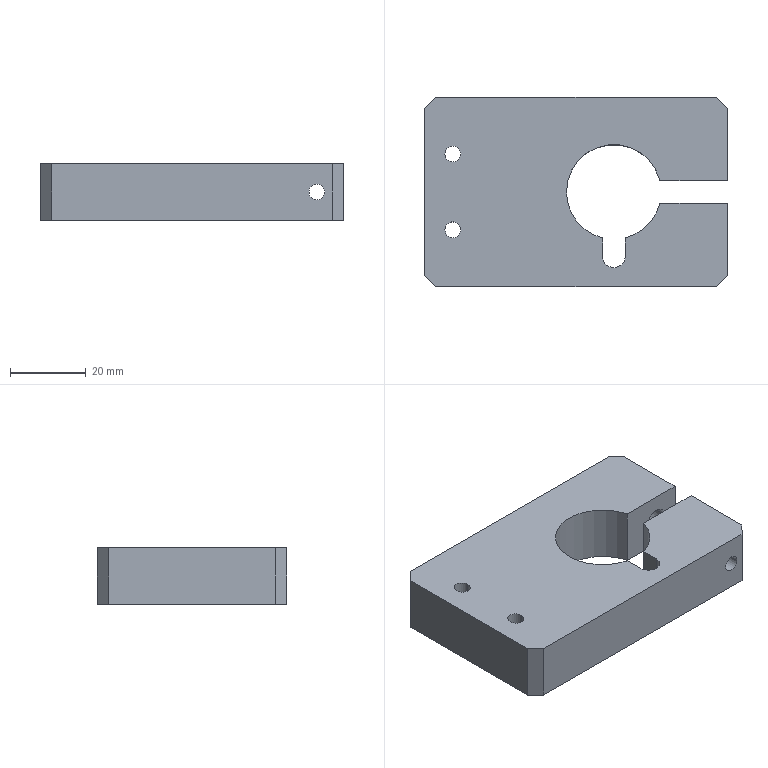Component | SolidWorks | 8TC-A15004-90-08A-1 | 1 solid | 31 faces | box 80 x 50 x 15 mm | volume 48295 mm3 | plane 16 | cylinder 15 | commonest cylinder face diameters 4.2 x6 25 x3 11 x2 6.6 x2 6 x2 | material A6061
STEP:
#1=CARTESIAN_POINT('',(-3.528,13.358,-1.969));
#2=VERTEX_POINT('',#1);
#3=CARTESIAN_POINT('',(-3.362,13.358,-1.969));
#4=VERTEX_POINT('',#3);
#5=CARTESIAN_POINT('',(-3.445,13.358,-1.969));
#6=DIRECTION('',(0.,0.,-1.));
#7=DIRECTION('',(1.,0.,0.));
#8=AXIS2_PLACEMENT_3D('',#5,#6,#7);
#9=CIRCLE('',#8,0.08268);
#10=EDGE_CURVE('',#2,#4,#9,.T.);
#11=ORIENTED_EDGE('',*,*,#10,.F.);
#12=CARTESIAN_POINT('',(-3.528,13.358,-2.559));
#13=VERTEX_POINT('',#12);
#14=CARTESIAN_POINT('',(-3.528,13.358,-2.559));
#15=DIRECTION('',(0.,0.,-1.));
#16=VECTOR('',#15,39.37);
#17=LINE('',#14,#16);
#18=EDGE_CURVE('',#2,#13,#17,.T.);
#19=ORIENTED_EDGE('',*,*,#18,.T.);
#20=CARTESIAN_POINT('',(-3.362,13.358,-2.559));
#21=VERTEX_POINT('',#20);
#22=CARTESIAN_POINT('',(-3.445,13.358,-2.559));
#23=DIRECTION('',(0.,0.,-1.));
#24=DIRECTION('',(1.,0.,0.));
#25=AXIS2_PLACEMENT_3D('',#22,#23,#24);
#26=CIRCLE('',#25,0.08268);
#27=EDGE_CURVE('',#13,#21,#26,.T.);
#28=ORIENTED_EDGE('',*,*,#27,.T.);
#29=CARTESIAN_POINT('',(-3.362,13.358,-2.559));
#30=DIRECTION('',(0.,0.,-1.));
#31=VECTOR('',#30,39.37);
#32=LINE('',#29,#31);
#33=EDGE_CURVE('',#4,#21,#32,.T.);
#34=ORIENTED_EDGE('',*,*,#33,.F.);
#35=EDGE_LOOP('',(#11,#19,#28,#34));
#36=FACE_OUTER_BOUND('',#35,.T.);
#37=CARTESIAN_POINT('',(-3.445,13.358,-2.559));
#38=DIRECTION('',(0.,0.,-1.));
#39=DIRECTION('',(1.,0.,0.));
#40=AXIS2_PLACEMENT_3D('',#37,#38,#39);
#41=CYLINDRICAL_SURFACE('',#40,0.08268);
#42=ADVANCED_FACE('',(#36),#41,.F.);
#43=CARTESIAN_POINT('',(-3.528,12.571,-1.969));
#44=VERTEX_POINT('',#43);
#45=CARTESIAN_POINT('',(-3.362,12.571,-1.969));
#46=VERTEX_POINT('',#45);
#47=CARTESIAN_POINT('',(-3.445,12.571,-1.969));
#48=DIRECTION('',(0.,0.,-1.));
#49=DIRECTION('',(1.,0.,0.));
#50=AXIS2_PLACEMENT_3D('',#47,#48,#49);
#51=CIRCLE('',#50,0.08268);
#52=EDGE_CURVE('',#44,#46,#51,.T.);
#53=ORIENTED_EDGE('',*,*,#52,.F.);
#54=CARTESIAN_POINT('',(-3.528,12.571,-2.559));
#55=VERTEX_POINT('',#54);
#56=CARTESIAN_POINT('',(-3.528,12.571,-2.559));
#57=DIRECTION('',(0.,0.,-1.));
#58=VECTOR('',#57,39.37);
#59=LINE('',#56,#58);
#60=EDGE_CURVE('',#44,#55,#59,.T.);
#61=ORIENTED_EDGE('',*,*,#60,.T.);
#62=CARTESIAN_POINT('',(-3.362,12.571,-2.559));
#63=VERTEX_POINT('',#62);
#64=CARTESIAN_POINT('',(-3.445,12.571,-2.559));
#65=DIRECTION('',(0.,0.,-1.));
#66=DIRECTION('',(1.,0.,0.));
#67=AXIS2_PLACEMENT_3D('',#64,#65,#66);
#68=CIRCLE('',#67,0.08268);
#69=EDGE_CURVE('',#55,#63,#68,.T.);
#70=ORIENTED_EDGE('',*,*,#69,.T.);
#71=CARTESIAN_POINT('',(-3.362,12.571,-2.559));
#72=DIRECTION('',(0.,0.,-1.));
#73=VECTOR('',#72,39.37);
#74=LINE('',#71,#73);
#75=EDGE_CURVE('',#46,#63,#74,.T.);
#76=ORIENTED_EDGE('',*,*,#75,.F.);
#77=EDGE_LOOP('',(#53,#61,#70,#76));
#78=FACE_OUTER_BOUND('',#77,.T.);
#79=CARTESIAN_POINT('',(-3.445,12.571,-2.559));
#80=DIRECTION('',(0.,0.,-1.));
#81=DIRECTION('',(1.,0.,0.));
#82=AXIS2_PLACEMENT_3D('',#79,#80,#81);
#83=CYLINDRICAL_SURFACE('',#82,0.08268);
#84=ADVANCED_FACE('',(#78),#83,.F.);
#85=CARTESIAN_POINT('',(-0.7835,11.98,-2.264));
#86=VERTEX_POINT('',#85);
#87=CARTESIAN_POINT('',(-0.9488,11.98,-2.264));
#88=VERTEX_POINT('',#87);
#89=CARTESIAN_POINT('',(-0.8661,11.98,-2.264));
#90=DIRECTION('',(-0.,1.,0.));
#91=DIRECTION('',(-1.,0.,0.));
#92=AXIS2_PLACEMENT_3D('',#89,#90,#91);
#93=CIRCLE('',#92,0.08268);
#94=EDGE_CURVE('',#86,#88,#93,.T.);
#95=ORIENTED_EDGE('',*,*,#94,.F.);
#96=CARTESIAN_POINT('',(-0.7835,12.846,-2.264));
#97=VERTEX_POINT('',#96);
#98=CARTESIAN_POINT('',(-0.7835,12.846,-2.264));
#99=DIRECTION('',(-0.,1.,0.));
#100=VECTOR('',#99,39.37);
#101=LINE('',#98,#100);
#102=EDGE_CURVE('',#86,#97,#101,.T.);
#103=ORIENTED_EDGE('',*,*,#102,.T.);
#104=CARTESIAN_POINT('',(-0.9488,12.846,-2.264));
#105=VERTEX_POINT('',#104);
#106=CARTESIAN_POINT('',(-0.8661,12.846,-2.264));
#107=DIRECTION('',(-0.,1.,0.));
#108=DIRECTION('',(-1.,0.,0.));
#109=AXIS2_PLACEMENT_3D('',#106,#107,#108);
#110=CIRCLE('',#109,0.08268);
#111=EDGE_CURVE('',#97,#105,#110,.T.);
#112=ORIENTED_EDGE('',*,*,#111,.T.);
#113=CARTESIAN_POINT('',(-0.9488,12.846,-2.264));
#114=DIRECTION('',(-0.,1.,0.));
#115=VECTOR('',#114,39.37);
#116=LINE('',#113,#115);
#117=EDGE_CURVE('',#88,#105,#116,.T.);
#118=ORIENTED_EDGE('',*,*,#117,.F.);
#119=EDGE_LOOP('',(#95,#103,#112,#118));
#120=FACE_OUTER_BOUND('',#119,.T.);
#121=CARTESIAN_POINT('',(-0.8661,12.846,-2.264));
#122=DIRECTION('',(-0.,1.,0.));
#123=DIRECTION('',(-1.,0.,0.));
#124=AXIS2_PLACEMENT_3D('',#121,#122,#123);
#125=CYLINDRICAL_SURFACE('',#124,0.08268);
#126=ADVANCED_FACE('',(#120),#125,.F.);
#127=CARTESIAN_POINT('',(-0.6496,13.697,-2.264));
#128=VERTEX_POINT('',#127);
#129=CARTESIAN_POINT('',(-1.083,13.697,-2.264));
#130=VERTEX_POINT('',#129);
#131=CARTESIAN_POINT('',(-0.8661,13.697,-2.264));
#132=DIRECTION('',(-0.,1.,0.));
#133=DIRECTION('',(-1.,0.,0.));
#134=AXIS2_PLACEMENT_3D('',#131,#132,#133);
#135=CIRCLE('',#134,0.2165);
#136=EDGE_CURVE('',#128,#130,#135,.T.);
#137=ORIENTED_EDGE('',*,*,#136,.F.);
#138=CARTESIAN_POINT('',(-0.6496,13.89,-2.264));
#139=VERTEX_POINT('',#138);
#140=CARTESIAN_POINT('',(-0.6496,13.949,-2.264));
#141=DIRECTION('',(-0.,1.,0.));
#142=VECTOR('',#141,39.37);
#143=LINE('',#140,#142);
#144=EDGE_CURVE('',#128,#139,#143,.T.);
#145=ORIENTED_EDGE('',*,*,#144,.T.);
#146=CARTESIAN_POINT('',(-0.7087,13.949,-2.412));
#147=VERTEX_POINT('',#146);
#148=CARTESIAN_POINT('',(-0.6496,13.89,-2.264));
#149=CARTESIAN_POINT('',(-0.6496,13.89,-2.32));
#150=CARTESIAN_POINT('',(-0.6703,13.91,-2.372));
#151=CARTESIAN_POINT('',(-0.7087,13.949,-2.412));
#152=(BOUNDED_CURVE()B_SPLINE_CURVE(3,(#148,#149,#150,#151),.UNSPECIFIED.,.F.,.F.)B_SPLINE_CURVE_WITH_KNOTS((4,4),(3.142,3.898),.UNSPECIFIED.)CURVE()GEOMETRIC_REPRESENTATION_ITEM()RATIONAL_B_SPLINE_CURVE((1.,0.9529,0.9529,1.))REPRESENTATION_ITEM(''));
#153=EDGE_CURVE('',#139,#147,#152,.T.);
#154=ORIENTED_EDGE('',*,*,#153,.T.);
#155=CARTESIAN_POINT('',(-1.083,13.949,-2.264));
#156=VERTEX_POINT('',#155);
#157=CARTESIAN_POINT('',(-0.8661,13.949,-2.264));
#158=DIRECTION('',(-0.,1.,0.));
#159=DIRECTION('',(-1.,0.,0.));
#160=AXIS2_PLACEMENT_3D('',#157,#158,#159);
#161=CIRCLE('',#160,0.2165);
#162=EDGE_CURVE('',#147,#156,#161,.T.);
#163=ORIENTED_EDGE('',*,*,#162,.T.);
#164=CARTESIAN_POINT('',(-1.083,13.949,-2.264));
#165=DIRECTION('',(-0.,1.,0.));
#166=VECTOR('',#165,39.37);
#167=LINE('',#164,#166);
#168=EDGE_CURVE('',#130,#156,#167,.T.);
#169=ORIENTED_EDGE('',*,*,#168,.F.);
#170=EDGE_LOOP('',(#137,#145,#154,#163,#169));
#171=FACE_OUTER_BOUND('',#170,.T.);
#172=CARTESIAN_POINT('',(-0.8661,13.949,-2.264));
#173=DIRECTION('',(-0.,1.,0.));
#174=DIRECTION('',(-1.,0.,0.));
#175=AXIS2_PLACEMENT_3D('',#172,#173,#174);
#176=CYLINDRICAL_SURFACE('',#175,0.2165);
#177=ADVANCED_FACE('',(#171),#176,.F.);
#178=CARTESIAN_POINT('',(-0.9961,13.083,-2.264));
#179=VERTEX_POINT('',#178);
#180=CARTESIAN_POINT('',(-0.7362,13.083,-2.264));
#181=VERTEX_POINT('',#180);
#182=CARTESIAN_POINT('',(-0.8661,13.083,-2.264));
#183=DIRECTION('',(-0.,-1.,-0.));
#184=DIRECTION('',(1.,0.,0.));
#185=AXIS2_PLACEMENT_3D('',#182,#183,#184);
#186=CIRCLE('',#185,0.1299);
#187=EDGE_CURVE('',#179,#181,#186,.T.);
#188=ORIENTED_EDGE('',*,*,#187,.T.);
#189=CARTESIAN_POINT('',(-0.7362,13.697,-2.264));
#190=VERTEX_POINT('',#189);
#191=CARTESIAN_POINT('',(-0.7362,13.949,-2.264));
#192=DIRECTION('',(-0.,1.,0.));
#193=VECTOR('',#192,39.37);
#194=LINE('',#191,#193);
#195=EDGE_CURVE('',#181,#190,#194,.T.);
#196=ORIENTED_EDGE('',*,*,#195,.T.);
#197=CARTESIAN_POINT('',(-0.9961,13.697,-2.264));
#198=VERTEX_POINT('',#197);
#199=CARTESIAN_POINT('',(-0.8661,13.697,-2.264));
#200=DIRECTION('',(-0.,1.,0.));
#201=DIRECTION('',(-1.,0.,0.));
#202=AXIS2_PLACEMENT_3D('',#199,#200,#201);
#203=CIRCLE('',#202,0.1299);
#204=EDGE_CURVE('',#190,#198,#203,.T.);
#205=ORIENTED_EDGE('',*,*,#204,.T.);
#206=CARTESIAN_POINT('',(-0.9961,13.949,-2.264));
#207=DIRECTION('',(-0.,1.,0.));
#208=VECTOR('',#207,39.37);
#209=LINE('',#206,#208);
#210=EDGE_CURVE('',#179,#198,#209,.T.);
#211=ORIENTED_EDGE('',*,*,#210,.F.);
#212=EDGE_LOOP('',(#188,#196,#205,#211));
#213=FACE_OUTER_BOUND('',#212,.T.);
#214=CARTESIAN_POINT('',(-0.8661,13.949,-2.264));
#215=DIRECTION('',(-0.,1.,0.));
#216=DIRECTION('',(-1.,0.,0.));
#217=AXIS2_PLACEMENT_3D('',#214,#215,#216);
#218=CYLINDRICAL_SURFACE('',#217,0.1299);
#219=ADVANCED_FACE('',(#213),#218,.F.);
#220=CARTESIAN_POINT('',(-1.89,12.487,-2.559));
#221=VERTEX_POINT('',#220);
#222=CARTESIAN_POINT('',(-2.264,12.965,-2.559));
#223=VERTEX_POINT('',#222);
#224=CARTESIAN_POINT('',(-1.772,12.965,-2.559));
#225=DIRECTION('',(0.,0.,-1.));
#226=DIRECTION('',(1.,0.,0.));
#227=AXIS2_PLACEMENT_3D('',#224,#225,#226);
#228=CIRCLE('',#227,0.4921);
#229=EDGE_CURVE('',#221,#223,#228,.T.);
#230=ORIENTED_EDGE('',*,*,#229,.T.);
#231=CARTESIAN_POINT('',(-2.264,12.965,-1.969));
#232=VERTEX_POINT('',#231);
#233=CARTESIAN_POINT('',(-2.264,12.965,-2.559));
#234=DIRECTION('',(-0.,-0.,1.));
#235=VECTOR('',#234,39.37);
#236=LINE('',#233,#235);
#237=EDGE_CURVE('',#223,#232,#236,.T.);
#238=ORIENTED_EDGE('',*,*,#237,.T.);
#239=CARTESIAN_POINT('',(-1.89,12.487,-1.969));
#240=VERTEX_POINT('',#239);
#241=CARTESIAN_POINT('',(-1.772,12.965,-1.969));
#242=DIRECTION('',(0.,0.,-1.));
#243=DIRECTION('',(1.,0.,0.));
#244=AXIS2_PLACEMENT_3D('',#241,#242,#243);
#245=CIRCLE('',#244,0.4921);
#246=EDGE_CURVE('',#240,#232,#245,.T.);
#247=ORIENTED_EDGE('',*,*,#246,.F.);
#248=CARTESIAN_POINT('',(-1.89,12.487,-1.969));
#249=DIRECTION('',(0.,0.,-1.));
#250=VECTOR('',#249,39.37);
#251=LINE('',#248,#250);
#252=EDGE_CURVE('',#240,#221,#251,.T.);
#253=ORIENTED_EDGE('',*,*,#252,.T.);
#254=EDGE_LOOP('',(#230,#238,#247,#253));
#255=FACE_OUTER_BOUND('',#254,.T.);
#256=CARTESIAN_POINT('',(-1.772,12.965,-2.559));
#257=DIRECTION('',(-0.,-0.,1.));
#258=DIRECTION('',(-1.,0.,0.));
#259=AXIS2_PLACEMENT_3D('',#256,#257,#258);
#260=CYLINDRICAL_SURFACE('',#259,0.4921);
#261=ADVANCED_FACE('',(#255),#260,.F.);
#262=ORIENTED_EDGE('',*,*,#162,.F.);
#263=CARTESIAN_POINT('',(-0.7087,13.949,-2.559));
#264=VERTEX_POINT('',#263);
#265=CARTESIAN_POINT('',(-0.7087,13.949,-2.264));
#266=DIRECTION('',(0.,0.,-1.));
#267=VECTOR('',#266,39.37);
#268=LINE('',#265,#267);
#269=EDGE_CURVE('',#147,#264,#268,.T.);
#270=ORIENTED_EDGE('',*,*,#269,.T.);
#271=CARTESIAN_POINT('',(-3.622,13.949,-2.559));
#272=VERTEX_POINT('',#271);
#273=CARTESIAN_POINT('',(-0.5906,13.949,-2.559));
#274=DIRECTION('',(1.,0.,0.));
#275=VECTOR('',#274,39.37);
#276=LINE('',#273,#275);
#277=EDGE_CURVE('',#272,#264,#276,.T.);
#278=ORIENTED_EDGE('',*,*,#277,.F.);
#279=CARTESIAN_POINT('',(-3.622,13.949,-1.969));
#280=VERTEX_POINT('',#279);
#281=CARTESIAN_POINT('',(-3.622,13.949,-2.264));
#282=DIRECTION('',(-0.,-0.,1.));
#283=VECTOR('',#282,39.37);
#284=LINE('',#281,#283);
#285=EDGE_CURVE('',#272,#280,#284,.T.);
#286=ORIENTED_EDGE('',*,*,#285,.T.);
#287=CARTESIAN_POINT('',(-0.7087,13.949,-1.969));
#288=VERTEX_POINT('',#287);
#289=CARTESIAN_POINT('',(-0.5906,13.949,-1.969));
#290=DIRECTION('',(-1.,-0.,-0.));
#291=VECTOR('',#290,39.37);
#292=LINE('',#289,#291);
#293=EDGE_CURVE('',#288,#280,#292,.T.);
#294=ORIENTED_EDGE('',*,*,#293,.F.);
#295=CARTESIAN_POINT('',(-0.7087,13.949,-2.115));
#296=VERTEX_POINT('',#295);
#297=CARTESIAN_POINT('',(-0.7087,13.949,-2.264));
#298=DIRECTION('',(0.,0.,-1.));
#299=VECTOR('',#298,39.37);
#300=LINE('',#297,#299);
#301=EDGE_CURVE('',#288,#296,#300,.T.);
#302=ORIENTED_EDGE('',*,*,#301,.T.);
#303=CARTESIAN_POINT('',(-0.8661,13.949,-2.264));
#304=DIRECTION('',(-0.,1.,0.));
#305=DIRECTION('',(-1.,0.,0.));
#306=AXIS2_PLACEMENT_3D('',#303,#304,#305);
#307=CIRCLE('',#306,0.2165);
#308=EDGE_CURVE('',#156,#296,#307,.T.);
#309=ORIENTED_EDGE('',*,*,#308,.F.);
#310=EDGE_LOOP('',(#262,#270,#278,#286,#294,#302,#309));
#311=FACE_OUTER_BOUND('',#310,.T.);
#312=CARTESIAN_POINT('',(-2.165,13.949,-2.264));
#313=DIRECTION('',(0.,-1.,-0.));
#314=DIRECTION('',(1.,0.,0.));
#315=AXIS2_PLACEMENT_3D('',#312,#313,#314);
#316=PLANE('',#315);
#317=ADVANCED_FACE('',(#311),#316,.F.);
#318=CARTESIAN_POINT('',(-1.654,12.487,-1.969));
#319=VERTEX_POINT('',#318);
#320=CARTESIAN_POINT('',(-1.654,12.487,-2.559));
#321=VERTEX_POINT('',#320);
#322=CARTESIAN_POINT('',(-1.654,12.487,-1.969));
#323=DIRECTION('',(0.,0.,-1.));
#324=VECTOR('',#323,39.37);
#325=LINE('',#322,#324);
#326=EDGE_CURVE('',#319,#321,#325,.T.);
#327=ORIENTED_EDGE('',*,*,#326,.F.);
#328=CARTESIAN_POINT('',(-1.294,12.846,-1.969));
#329=VERTEX_POINT('',#328);
#330=CARTESIAN_POINT('',(-1.772,12.965,-1.969));
#331=DIRECTION('',(0.,0.,-1.));
#332=DIRECTION('',(1.,0.,0.));
#333=AXIS2_PLACEMENT_3D('',#330,#331,#332);
#334=CIRCLE('',#333,0.4921);
#335=EDGE_CURVE('',#329,#319,#334,.T.);
#336=ORIENTED_EDGE('',*,*,#335,.F.);
#337=CARTESIAN_POINT('',(-1.294,12.846,-2.559));
#338=VERTEX_POINT('',#337);
#339=CARTESIAN_POINT('',(-1.294,12.846,-2.559));
#340=DIRECTION('',(-0.,-0.,1.));
#341=VECTOR('',#340,39.37);
#342=LINE('',#339,#341);
#343=EDGE_CURVE('',#338,#329,#342,.T.);
#344=ORIENTED_EDGE('',*,*,#343,.F.);
#345=CARTESIAN_POINT('',(-1.772,12.965,-2.559));
#346=DIRECTION('',(0.,0.,-1.));
#347=DIRECTION('',(1.,0.,0.));
#348=AXIS2_PLACEMENT_3D('',#345,#346,#347);
#349=CIRCLE('',#348,0.4921);
#350=EDGE_CURVE('',#338,#321,#349,.T.);
#351=ORIENTED_EDGE('',*,*,#350,.T.);
#352=EDGE_LOOP('',(#327,#336,#344,#351));
#353=FACE_OUTER_BOUND('',#352,.T.);
#354=CARTESIAN_POINT('',(-1.772,12.965,-2.559));
#355=DIRECTION('',(-0.,-0.,1.));
#356=DIRECTION('',(-1.,0.,0.));
#357=AXIS2_PLACEMENT_3D('',#354,#355,#356);
#358=CYLINDRICAL_SURFACE('',#357,0.4921);
#359=ADVANCED_FACE('',(#353),#358,.F.);
#360=CARTESIAN_POINT('',(-3.445,13.358,-2.559));
#361=DIRECTION('',(0.,0.,-1.));
#362=DIRECTION('',(1.,0.,0.));
#363=AXIS2_PLACEMENT_3D('',#360,#361,#362);
#364=CIRCLE('',#363,0.08268);
#365=EDGE_CURVE('',#21,#13,#364,.T.);
#366=ORIENTED_EDGE('',*,*,#365,.F.);
#367=ORIENTED_EDGE('',*,*,#27,.F.);
#368=EDGE_LOOP('',(#366,#367));
#369=FACE_BOUND('',#368,.T.);
#370=CARTESIAN_POINT('',(-3.445,12.571,-2.559));
#371=DIRECTION('',(0.,0.,-1.));
#372=DIRECTION('',(1.,0.,0.));
#373=AXIS2_PLACEMENT_3D('',#370,#371,#372);
#374=CIRCLE('',#373,0.08268);
#375=EDGE_CURVE('',#63,#55,#374,.T.);
#376=ORIENTED_EDGE('',*,*,#375,.F.);
#377=ORIENTED_EDGE('',*,*,#69,.F.);
#378=EDGE_LOOP('',(#376,#377));
#379=FACE_BOUND('',#378,.T.);
#380=CARTESIAN_POINT('',(-3.622,11.98,-2.559));
#381=VERTEX_POINT('',#380);
#382=CARTESIAN_POINT('',(-0.7087,11.98,-2.559));
#383=VERTEX_POINT('',#382);
#384=CARTESIAN_POINT('',(-0.5906,11.98,-2.559));
#385=DIRECTION('',(1.,0.,0.));
#386=VECTOR('',#385,39.37);
#387=LINE('',#384,#386);
#388=EDGE_CURVE('',#381,#383,#387,.T.);
#389=ORIENTED_EDGE('',*,*,#388,.F.);
#390=CARTESIAN_POINT('',(-3.74,12.098,-2.559));
#391=VERTEX_POINT('',#390);
#392=CARTESIAN_POINT('',(-3.622,11.98,-2.559));
#393=DIRECTION('',(-0.7071,0.7071,0.));
#394=VECTOR('',#393,39.37);
#395=LINE('',#392,#394);
#396=EDGE_CURVE('',#381,#391,#395,.T.);
#397=ORIENTED_EDGE('',*,*,#396,.T.);
#398=CARTESIAN_POINT('',(-3.74,13.831,-2.559));
#399=VERTEX_POINT('',#398);
#400=CARTESIAN_POINT('',(-3.74,11.98,-2.559));
#401=DIRECTION('',(-0.,1.,0.));
#402=VECTOR('',#401,39.37);
#403=LINE('',#400,#402);
#404=EDGE_CURVE('',#391,#399,#403,.T.);
#405=ORIENTED_EDGE('',*,*,#404,.T.);
#406=CARTESIAN_POINT('',(-3.74,13.831,-2.559));
#407=DIRECTION('',(0.7071,0.7071,0.));
#408=VECTOR('',#407,39.37);
#409=LINE('',#406,#408);
#410=EDGE_CURVE('',#399,#272,#409,.T.);
#411=ORIENTED_EDGE('',*,*,#410,.T.);
#412=ORIENTED_EDGE('',*,*,#277,.T.);
#413=CARTESIAN_POINT('',(-0.5906,13.831,-2.559));
#414=VERTEX_POINT('',#413);
#415=CARTESIAN_POINT('',(-0.5906,13.831,-2.559));
#416=DIRECTION('',(0.7071,-0.7071,-0.));
#417=VECTOR('',#416,39.37);
#418=LINE('',#415,#417);
#419=EDGE_CURVE('',#264,#414,#418,.T.);
#420=ORIENTED_EDGE('',*,*,#419,.T.);
#421=CARTESIAN_POINT('',(-0.5906,13.083,-2.559));
#422=VERTEX_POINT('',#421);
#423=CARTESIAN_POINT('',(-0.5906,11.98,-2.559));
#424=DIRECTION('',(-0.,1.,0.));
#425=VECTOR('',#424,39.37);
#426=LINE('',#423,#425);
#427=EDGE_CURVE('',#422,#414,#426,.T.);
#428=ORIENTED_EDGE('',*,*,#427,.F.);
#429=CARTESIAN_POINT('',(-1.294,13.083,-2.559));
#430=VERTEX_POINT('',#429);
#431=CARTESIAN_POINT('',(-0.5906,13.083,-2.559));
#432=DIRECTION('',(1.,-0.,0.));
#433=VECTOR('',#432,39.37);
#434=LINE('',#431,#433);
#435=EDGE_CURVE('',#430,#422,#434,.T.);
#436=ORIENTED_EDGE('',*,*,#435,.F.);
#437=CARTESIAN_POINT('',(-1.772,12.965,-2.559));
#438=DIRECTION('',(0.,0.,-1.));
#439=DIRECTION('',(1.,0.,0.));
#440=AXIS2_PLACEMENT_3D('',#437,#438,#439);
#441=CIRCLE('',#440,0.4921);
#442=EDGE_CURVE('',#223,#430,#441,.T.);
#443=ORIENTED_EDGE('',*,*,#442,.F.);
#444=ORIENTED_EDGE('',*,*,#229,.F.);
#445=CARTESIAN_POINT('',(-1.89,12.295,-2.559));
#446=VERTEX_POINT('',#445);
#447=CARTESIAN_POINT('',(-1.89,12.487,-2.559));
#448=DIRECTION('',(-0.,1.,0.));
#449=VECTOR('',#448,39.37);
#450=LINE('',#447,#449);
#451=EDGE_CURVE('',#446,#221,#450,.T.);
#452=ORIENTED_EDGE('',*,*,#451,.F.);
#453=CARTESIAN_POINT('',(-1.772,12.177,-2.559));
#454=VERTEX_POINT('',#453);
#455=CARTESIAN_POINT('',(-1.772,12.295,-2.559));
#456=DIRECTION('',(-0.,-0.,1.));
#457=DIRECTION('',(-1.,0.,0.));
#458=AXIS2_PLACEMENT_3D('',#455,#456,#457);
#459=CIRCLE('',#458,0.1181);
#460=EDGE_CURVE('',#446,#454,#459,.T.);
#461=ORIENTED_EDGE('',*,*,#460,.T.);
#462=CARTESIAN_POINT('',(-1.654,12.295,-2.559));
#463=VERTEX_POINT('',#462);
#464=CARTESIAN_POINT('',(-1.772,12.295,-2.559));
#465=DIRECTION('',(-0.,-0.,1.));
#466=DIRECTION('',(-1.,0.,0.));
#467=AXIS2_PLACEMENT_3D('',#464,#465,#466);
#468=CIRCLE('',#467,0.1181);
#469=EDGE_CURVE('',#454,#463,#468,.T.);
#470=ORIENTED_EDGE('',*,*,#469,.T.);
#471=CARTESIAN_POINT('',(-1.654,12.487,-2.559));
#472=DIRECTION('',(0.,-1.,-0.));
#473=VECTOR('',#472,39.37);
#474=LINE('',#471,#473);
#475=EDGE_CURVE('',#321,#463,#474,.T.);
#476=ORIENTED_EDGE('',*,*,#475,.F.);
#477=ORIENTED_EDGE('',*,*,#350,.F.);
#478=CARTESIAN_POINT('',(-0.5906,12.846,-2.559));
#479=VERTEX_POINT('',#478);
#480=CARTESIAN_POINT('',(-0.5906,12.846,-2.559));
#481=DIRECTION('',(-1.,0.,-0.));
#482=VECTOR('',#481,39.37);
#483=LINE('',#480,#482);
#484=EDGE_CURVE('',#479,#338,#483,.T.);
#485=ORIENTED_EDGE('',*,*,#484,.F.);
#486=CARTESIAN_POINT('',(-0.5906,12.098,-2.559));
#487=VERTEX_POINT('',#486);
#488=CARTESIAN_POINT('',(-0.5906,11.98,-2.559));
#489=DIRECTION('',(-0.,1.,0.));
#490=VECTOR('',#489,39.37);
#491=LINE('',#488,#490);
#492=EDGE_CURVE('',#487,#479,#491,.T.);
#493=ORIENTED_EDGE('',*,*,#492,.F.);
#494=CARTESIAN_POINT('',(-0.7087,11.98,-2.559));
#495=DIRECTION('',(-0.7071,-0.7071,-0.));
#496=VECTOR('',#495,39.37);
#497=LINE('',#494,#496);
#498=EDGE_CURVE('',#487,#383,#497,.T.);
#499=ORIENTED_EDGE('',*,*,#498,.T.);
#500=EDGE_LOOP('',(#389,#397,#405,#411,#412,#420,#428,#436,#443,#444,#452,#461,#470,#476,#477,#485,#493,#499));
#501=FACE_OUTER_BOUND('',#500,.T.);
#502=CARTESIAN_POINT('',(-0.5906,11.98,-2.559));
#503=DIRECTION('',(-0.,-0.,1.));
#504=DIRECTION('',(-1.,-0.,-0.));
#505=AXIS2_PLACEMENT_3D('',#502,#503,#504);
#506=PLANE('',#505);
#507=ADVANCED_FACE('',(#369,#379,#501),#506,.F.);
#508=ORIENTED_EDGE('',*,*,#427,.T.);
#509=CARTESIAN_POINT('',(-0.5906,13.831,-1.969));
#510=VERTEX_POINT('',#509);
#511=CARTESIAN_POINT('',(-0.5906,13.831,-2.559));
#512=DIRECTION('',(-0.,-0.,1.));
#513=VECTOR('',#512,39.37);
#514=LINE('',#511,#513);
#515=EDGE_CURVE('',#414,#510,#514,.T.);
#516=ORIENTED_EDGE('',*,*,#515,.T.);
#517=CARTESIAN_POINT('',(-0.5906,13.083,-1.969));
#518=VERTEX_POINT('',#517);
#519=CARTESIAN_POINT('',(-0.5906,11.98,-1.969));
#520=DIRECTION('',(-0.,1.,0.));
#521=VECTOR('',#520,39.37);
#522=LINE('',#519,#521);
#523=EDGE_CURVE('',#518,#510,#522,.T.);
#524=ORIENTED_EDGE('',*,*,#523,.F.);
#525=CARTESIAN_POINT('',(-0.5906,13.083,-2.559));
#526=DIRECTION('',(-0.,-0.,1.));
#527=VECTOR('',#526,39.37);
#528=LINE('',#525,#527);
#529=EDGE_CURVE('',#422,#518,#528,.T.);
#530=ORIENTED_EDGE('',*,*,#529,.F.);
#531=EDGE_LOOP('',(#508,#516,#524,#530));
#532=FACE_OUTER_BOUND('',#531,.T.);
#533=CARTESIAN_POINT('',(-0.5906,11.98,-2.559));
#534=DIRECTION('',(-1.,-0.,-0.));
#535=DIRECTION('',(0.,0.,-1.));
#536=AXIS2_PLACEMENT_3D('',#533,#534,#535);
#537=PLANE('',#536);
#538=ADVANCED_FACE('',(#532),#537,.F.);
#539=CARTESIAN_POINT('',(-0.5906,12.098,-1.969));
#540=VERTEX_POINT('',#539);
#541=CARTESIAN_POINT('',(-0.5906,12.846,-1.969));
#542=VERTEX_POINT('',#541);
#543=CARTESIAN_POINT('',(-0.5906,11.98,-1.969));
#544=DIRECTION('',(-0.,1.,0.));
#545=VECTOR('',#544,39.37);
#546=LINE('',#543,#545);
#547=EDGE_CURVE('',#540,#542,#546,.T.);
#548=ORIENTED_EDGE('',*,*,#547,.F.);
#549=CARTESIAN_POINT('',(-0.5906,12.098,-2.559));
#550=DIRECTION('',(0.,0.,-1.));
#551=VECTOR('',#550,39.37);
#552=LINE('',#549,#551);
#553=EDGE_CURVE('',#540,#487,#552,.T.);
#554=ORIENTED_EDGE('',*,*,#553,.T.);
#555=ORIENTED_EDGE('',*,*,#492,.T.);
#556=CARTESIAN_POINT('',(-0.5906,12.846,-2.559));
#557=DIRECTION('',(-0.,-0.,1.));
#558=VECTOR('',#557,39.37);
#559=LINE('',#556,#558);
#560=EDGE_CURVE('',#479,#542,#559,.T.);
#561=ORIENTED_EDGE('',*,*,#560,.T.);
#562=EDGE_LOOP('',(#548,#554,#555,#561));
#563=FACE_OUTER_BOUND('',#562,.T.);
#564=CARTESIAN_POINT('',(-0.5906,11.98,-2.559));
#565=DIRECTION('',(-1.,-0.,-0.));
#566=DIRECTION('',(0.,0.,-1.));
#567=AXIS2_PLACEMENT_3D('',#564,#565,#566);
#568=PLANE('',#567);
#569=ADVANCED_FACE('',(#563),#568,.F.);
#570=CARTESIAN_POINT('',(-3.445,13.358,-1.969));
#571=DIRECTION('',(0.,0.,-1.));
#572=DIRECTION('',(1.,0.,0.));
#573=AXIS2_PLACEMENT_3D('',#570,#571,#572);
#574=CIRCLE('',#573,0.08268);
#575=EDGE_CURVE('',#4,#2,#574,.T.);
#576=ORIENTED_EDGE('',*,*,#575,.T.);
#577=ORIENTED_EDGE('',*,*,#10,.T.);
#578=EDGE_LOOP('',(#576,#577));
#579=FACE_BOUND('',#578,.T.);
#580=CARTESIAN_POINT('',(-3.445,12.571,-1.969));
#581=DIRECTION('',(0.,0.,-1.));
#582=DIRECTION('',(1.,0.,0.));
#583=AXIS2_PLACEMENT_3D('',#580,#581,#582);
#584=CIRCLE('',#583,0.08268);
#585=EDGE_CURVE('',#46,#44,#584,.T.);
#586=ORIENTED_EDGE('',*,*,#585,.T.);
#587=ORIENTED_EDGE('',*,*,#52,.T.);
#588=EDGE_LOOP('',(#586,#587));
#589=FACE_BOUND('',#588,.T.);
#590=CARTESIAN_POINT('',(-3.74,12.098,-1.969));
#591=VERTEX_POINT('',#590);
#592=CARTESIAN_POINT('',(-3.74,13.831,-1.969));
#593=VERTEX_POINT('',#592);
#594=CARTESIAN_POINT('',(-3.74,11.98,-1.969));
#595=DIRECTION('',(-0.,1.,0.));
#596=VECTOR('',#595,39.37);
#597=LINE('',#594,#596);
#598=EDGE_CURVE('',#591,#593,#597,.T.);
#599=ORIENTED_EDGE('',*,*,#598,.F.);
#600=CARTESIAN_POINT('',(-3.622,11.98,-1.969));
#601=VERTEX_POINT('',#600);
#602=CARTESIAN_POINT('',(-3.622,11.98,-1.969));
#603=DIRECTION('',(0.7071,-0.7071,-0.));
#604=VECTOR('',#603,39.37);
#605=LINE('',#602,#604);
#606=EDGE_CURVE('',#591,#601,#605,.T.);
#607=ORIENTED_EDGE('',*,*,#606,.T.);
#608=CARTESIAN_POINT('',(-0.7087,11.98,-1.969));
#609=VERTEX_POINT('',#608);
#610=CARTESIAN_POINT('',(-0.5906,11.98,-1.969));
#611=DIRECTION('',(-1.,-0.,-0.));
#612=VECTOR('',#611,39.37);
#613=LINE('',#610,#612);
#614=EDGE_CURVE('',#609,#601,#613,.T.);
#615=ORIENTED_EDGE('',*,*,#614,.F.);
#616=CARTESIAN_POINT('',(-0.7087,11.98,-1.969));
#617=DIRECTION('',(0.7071,0.7071,0.));
#618=VECTOR('',#617,39.37);
#619=LINE('',#616,#618);
#620=EDGE_CURVE('',#609,#540,#619,.T.);
#621=ORIENTED_EDGE('',*,*,#620,.T.);
#622=ORIENTED_EDGE('',*,*,#547,.T.);
#623=CARTESIAN_POINT('',(-0.5906,12.846,-1.969));
#624=DIRECTION('',(-1.,0.,-0.));
#625=VECTOR('',#624,39.37);
#626=LINE('',#623,#625);
#627=EDGE_CURVE('',#542,#329,#626,.T.);
#628=ORIENTED_EDGE('',*,*,#627,.T.);
#629=ORIENTED_EDGE('',*,*,#335,.T.);
#630=CARTESIAN_POINT('',(-1.654,12.295,-1.969));
#631=VERTEX_POINT('',#630);
#632=CARTESIAN_POINT('',(-1.654,12.487,-1.969));
#633=DIRECTION('',(0.,-1.,-0.));
#634=VECTOR('',#633,39.37);
#635=LINE('',#632,#634);
#636=EDGE_CURVE('',#319,#631,#635,.T.);
#637=ORIENTED_EDGE('',*,*,#636,.T.);
#638=CARTESIAN_POINT('',(-1.772,12.177,-1.969));
#639=VERTEX_POINT('',#638);
#640=CARTESIAN_POINT('',(-1.772,12.295,-1.969));
#641=DIRECTION('',(0.,0.,-1.));
#642=DIRECTION('',(1.,0.,0.));
#643=AXIS2_PLACEMENT_3D('',#640,#641,#642);
#644=CIRCLE('',#643,0.1181);
#645=EDGE_CURVE('',#631,#639,#644,.T.);
#646=ORIENTED_EDGE('',*,*,#645,.T.);
#647=CARTESIAN_POINT('',(-1.89,12.295,-1.969));
#648=VERTEX_POINT('',#647);
#649=CARTESIAN_POINT('',(-1.772,12.295,-1.969));
#650=DIRECTION('',(0.,0.,-1.));
#651=DIRECTION('',(1.,0.,0.));
#652=AXIS2_PLACEMENT_3D('',#649,#650,#651);
#653=CIRCLE('',#652,0.1181);
#654=EDGE_CURVE('',#639,#648,#653,.T.);
#655=ORIENTED_EDGE('',*,*,#654,.T.);
#656=CARTESIAN_POINT('',(-1.89,12.487,-1.969));
#657=DIRECTION('',(-0.,1.,0.));
#658=VECTOR('',#657,39.37);
#659=LINE('',#656,#658);
#660=EDGE_CURVE('',#648,#240,#659,.T.);
#661=ORIENTED_EDGE('',*,*,#660,.T.);
#662=ORIENTED_EDGE('',*,*,#246,.T.);
#663=CARTESIAN_POINT('',(-1.294,13.083,-1.969));
#664=VERTEX_POINT('',#663);
#665=CARTESIAN_POINT('',(-1.772,12.965,-1.969));
#666=DIRECTION('',(0.,0.,-1.));
#667=DIRECTION('',(1.,0.,0.));
#668=AXIS2_PLACEMENT_3D('',#665,#666,#667);
#669=CIRCLE('',#668,0.4921);
#670=EDGE_CURVE('',#232,#664,#669,.T.);
#671=ORIENTED_EDGE('',*,*,#670,.T.);
#672=CARTESIAN_POINT('',(-0.5906,13.083,-1.969));
#673=DIRECTION('',(1.,-0.,0.));
#674=VECTOR('',#673,39.37);
#675=LINE('',#672,#674);
#676=EDGE_CURVE('',#664,#518,#675,.T.);
#677=ORIENTED_EDGE('',*,*,#676,.T.);
#678=ORIENTED_EDGE('',*,*,#523,.T.);
#679=CARTESIAN_POINT('',(-0.5906,13.831,-1.969));
#680=DIRECTION('',(-0.7071,0.7071,0.));
#681=VECTOR('',#680,39.37);
#682=LINE('',#679,#681);
#683=EDGE_CURVE('',#510,#288,#682,.T.);
#684=ORIENTED_EDGE('',*,*,#683,.T.);
#685=ORIENTED_EDGE('',*,*,#293,.T.);
#686=CARTESIAN_POINT('',(-3.74,13.831,-1.969));
#687=DIRECTION('',(-0.7071,-0.7071,-0.));
#688=VECTOR('',#687,39.37);
#689=LINE('',#686,#688);
#690=EDGE_CURVE('',#280,#593,#689,.T.);
#691=ORIENTED_EDGE('',*,*,#690,.T.);
#692=EDGE_LOOP('',(#599,#607,#615,#621,#622,#628,#629,#637,#646,#655,#661,#662,#671,#677,#678,#684,#685,#691));
#693=FACE_OUTER_BOUND('',#692,.T.);
#694=CARTESIAN_POINT('',(-0.5906,11.98,-1.969));
#695=DIRECTION('',(0.,0.,-1.));
#696=DIRECTION('',(1.,0.,0.));
#697=AXIS2_PLACEMENT_3D('',#694,#695,#696);
#698=PLANE('',#697);
#699=ADVANCED_FACE('',(#579,#589,#693),#698,.F.);
#700=ORIENTED_EDGE('',*,*,#237,.F.);
#701=ORIENTED_EDGE('',*,*,#442,.T.);
#702=CARTESIAN_POINT('',(-1.294,13.083,-2.559));
#703=DIRECTION('',(-0.,-0.,1.));
#704=VECTOR('',#703,39.37);
#705=LINE('',#702,#704);
#706=EDGE_CURVE('',#430,#664,#705,.T.);
#707=ORIENTED_EDGE('',*,*,#706,.T.);
#708=ORIENTED_EDGE('',*,*,#670,.F.);
#709=EDGE_LOOP('',(#700,#701,#707,#708));
#710=FACE_OUTER_BOUND('',#709,.T.);
#711=CARTESIAN_POINT('',(-1.772,12.965,-2.559));
#712=DIRECTION('',(-0.,-0.,1.));
#713=DIRECTION('',(-1.,0.,0.));
#714=AXIS2_PLACEMENT_3D('',#711,#712,#713);
#715=CYLINDRICAL_SURFACE('',#714,0.4921);
#716=ADVANCED_FACE('',(#710),#715,.F.);
#717=ORIENTED_EDGE('',*,*,#404,.F.);
#718=CARTESIAN_POINT('',(-3.74,12.098,-1.969));
#719=DIRECTION('',(-0.,-0.,1.));
#720=VECTOR('',#719,39.37);
#721=LINE('',#718,#720);
#722=EDGE_CURVE('',#391,#591,#721,.T.);
#723=ORIENTED_EDGE('',*,*,#722,.T.);
#724=ORIENTED_EDGE('',*,*,#598,.T.);
#725=CARTESIAN_POINT('',(-3.74,13.831,-2.559));
#726=DIRECTION('',(0.,0.,-1.));
#727=VECTOR('',#726,39.37);
#728=LINE('',#725,#727);
#729=EDGE_CURVE('',#593,#399,#728,.T.);
#730=ORIENTED_EDGE('',*,*,#729,.T.);
#731=EDGE_LOOP('',(#717,#723,#724,#730));
#732=FACE_OUTER_BOUND('',#731,.T.);
#733=CARTESIAN_POINT('',(-3.74,11.98,-2.559));
#734=DIRECTION('',(1.,0.,0.));
#735=DIRECTION('',(-0.,-0.,1.));
#736=AXIS2_PLACEMENT_3D('',#733,#734,#735);
#737=PLANE('',#736);
#738=ADVANCED_FACE('',(#732),#737,.F.);
#739=CARTESIAN_POINT('',(-0.8661,11.98,-2.264));
#740=DIRECTION('',(-0.,1.,0.));
#741=DIRECTION('',(-1.,0.,0.));
#742=AXIS2_PLACEMENT_3D('',#739,#740,#741);
#743=CIRCLE('',#742,0.08268);
#744=EDGE_CURVE('',#88,#86,#743,.T.);
#745=ORIENTED_EDGE('',*,*,#744,.T.);
#746=ORIENTED_EDGE('',*,*,#94,.T.);
#747=EDGE_LOOP('',(#745,#746));
#748=FACE_BOUND('',#747,.T.);
#749=ORIENTED_EDGE('',*,*,#614,.T.);
#750=CARTESIAN_POINT('',(-3.622,11.98,-2.559));
#751=DIRECTION('',(0.,0.,-1.));
#752=VECTOR('',#751,39.37);
#753=LINE('',#750,#752);
#754=EDGE_CURVE('',#601,#381,#753,.T.);
#755=ORIENTED_EDGE('',*,*,#754,.T.);
#756=ORIENTED_EDGE('',*,*,#388,.T.);
#757=CARTESIAN_POINT('',(-0.7087,11.98,-1.969));
#758=DIRECTION('',(-0.,-0.,1.));
#759=VECTOR('',#758,39.37);
#760=LINE('',#757,#759);
#761=EDGE_CURVE('',#383,#609,#760,.T.);
#762=ORIENTED_EDGE('',*,*,#761,.T.);
#763=EDGE_LOOP('',(#749,#755,#756,#762));
#764=FACE_OUTER_BOUND('',#763,.T.);
#765=CARTESIAN_POINT('',(-2.165,11.98,-2.264));
#766=DIRECTION('',(0.,-1.,-0.));
#767=DIRECTION('',(1.,0.,0.));
#768=AXIS2_PLACEMENT_3D('',#765,#766,#767);
#769=PLANE('',#768);
#770=ADVANCED_FACE('',(#748,#764),#769,.T.);
#771=CARTESIAN_POINT('',(-0.8661,12.846,-2.264));
#772=DIRECTION('',(-0.,1.,0.));
#773=DIRECTION('',(-1.,0.,0.));
#774=AXIS2_PLACEMENT_3D('',#771,#772,#773);
#775=CIRCLE('',#774,0.08268);
#776=EDGE_CURVE('',#105,#97,#775,.T.);
#777=ORIENTED_EDGE('',*,*,#776,.F.);
#778=ORIENTED_EDGE('',*,*,#111,.F.);
#779=EDGE_LOOP('',(#777,#778));
#780=FACE_BOUND('',#779,.T.);
#781=ORIENTED_EDGE('',*,*,#627,.F.);
#782=ORIENTED_EDGE('',*,*,#560,.F.);
#783=ORIENTED_EDGE('',*,*,#484,.T.);
#784=ORIENTED_EDGE('',*,*,#343,.T.);
#785=EDGE_LOOP('',(#781,#782,#783,#784));
#786=FACE_OUTER_BOUND('',#785,.T.);
#787=CARTESIAN_POINT('',(-0.5906,12.846,-2.559));
#788=DIRECTION('',(0.,1.,0.));
#789=DIRECTION('',(-1.,0.,-0.));
#790=AXIS2_PLACEMENT_3D('',#787,#788,#789);
#791=PLANE('',#790);
#792=ADVANCED_FACE('',(#780,#786),#791,.T.);
#793=ORIENTED_EDGE('',*,*,#187,.F.);
#794=CARTESIAN_POINT('',(-0.8661,13.083,-2.264));
#795=DIRECTION('',(-0.,-1.,-0.));
#796=DIRECTION('',(1.,0.,0.));
#797=AXIS2_PLACEMENT_3D('',#794,#795,#796);
#798=CIRCLE('',#797,0.1299);
#799=EDGE_CURVE('',#181,#179,#798,.T.);
#800=ORIENTED_EDGE('',*,*,#799,.F.);
#801=EDGE_LOOP('',(#793,#800));
#802=FACE_BOUND('',#801,.T.);
#803=ORIENTED_EDGE('',*,*,#676,.F.);
#804=ORIENTED_EDGE('',*,*,#706,.F.);
#805=ORIENTED_EDGE('',*,*,#435,.T.);
#806=ORIENTED_EDGE('',*,*,#529,.T.);
#807=EDGE_LOOP('',(#803,#804,#805,#806));
#808=FACE_OUTER_BOUND('',#807,.T.);
#809=CARTESIAN_POINT('',(-0.5906,13.083,-2.559));
#810=DIRECTION('',(-0.,-1.,-0.));
#811=DIRECTION('',(1.,-0.,0.));
#812=AXIS2_PLACEMENT_3D('',#809,#810,#811);
#813=PLANE('',#812);
#814=ADVANCED_FACE('',(#802,#808),#813,.T.);
#815=ORIENTED_EDGE('',*,*,#475,.T.);
#816=CARTESIAN_POINT('',(-1.654,12.295,-1.969));
#817=DIRECTION('',(-0.,-0.,1.));
#818=VECTOR('',#817,39.37);
#819=LINE('',#816,#818);
#820=EDGE_CURVE('',#463,#631,#819,.T.);
#821=ORIENTED_EDGE('',*,*,#820,.T.);
#822=ORIENTED_EDGE('',*,*,#636,.F.);
#823=ORIENTED_EDGE('',*,*,#326,.T.);
#824=EDGE_LOOP('',(#815,#821,#822,#823));
#825=FACE_OUTER_BOUND('',#824,.T.);
#826=CARTESIAN_POINT('',(-1.654,12.487,-1.969));
#827=DIRECTION('',(1.,0.,0.));
#828=DIRECTION('',(-0.,-0.,1.));
#829=AXIS2_PLACEMENT_3D('',#826,#827,#828);
#830=PLANE('',#829);
#831=ADVANCED_FACE('',(#825),#830,.F.);
#832=ORIENTED_EDGE('',*,*,#660,.F.);
#833=CARTESIAN_POINT('',(-1.89,12.295,-2.559));
#834=DIRECTION('',(0.,0.,-1.));
#835=VECTOR('',#834,39.37);
#836=LINE('',#833,#835);
#837=EDGE_CURVE('',#648,#446,#836,.T.);
#838=ORIENTED_EDGE('',*,*,#837,.T.);
#839=ORIENTED_EDGE('',*,*,#451,.T.);
#840=ORIENTED_EDGE('',*,*,#252,.F.);
#841=EDGE_LOOP('',(#832,#838,#839,#840));
#842=FACE_OUTER_BOUND('',#841,.T.);
#843=CARTESIAN_POINT('',(-1.89,12.487,-1.969));
#844=DIRECTION('',(-1.,-0.,-0.));
#845=DIRECTION('',(0.,0.,-1.));
#846=AXIS2_PLACEMENT_3D('',#843,#844,#845);
#847=PLANE('',#846);
#848=ADVANCED_FACE('',(#842),#847,.F.);
#849=ORIENTED_EDGE('',*,*,#606,.F.);
#850=ORIENTED_EDGE('',*,*,#722,.F.);
#851=ORIENTED_EDGE('',*,*,#396,.F.);
#852=ORIENTED_EDGE('',*,*,#754,.F.);
#853=EDGE_LOOP('',(#849,#850,#851,#852));
#854=FACE_OUTER_BOUND('',#853,.T.);
#855=CARTESIAN_POINT('',(-3.622,11.98,-2.264));
#856=DIRECTION('',(-0.7071,-0.7071,-0.));
#857=DIRECTION('',(-0.,-0.,1.));
#858=AXIS2_PLACEMENT_3D('',#855,#856,#857);
#859=PLANE('',#858);
#860=ADVANCED_FACE('',(#854),#859,.T.);
#861=ORIENTED_EDGE('',*,*,#690,.F.);
#862=ORIENTED_EDGE('',*,*,#285,.F.);
#863=ORIENTED_EDGE('',*,*,#410,.F.);
#864=ORIENTED_EDGE('',*,*,#729,.F.);
#865=EDGE_LOOP('',(#861,#862,#863,#864));
#866=FACE_OUTER_BOUND('',#865,.T.);
#867=CARTESIAN_POINT('',(-3.74,13.831,-2.559));
#868=DIRECTION('',(0.7071,-0.7071,-0.));
#869=DIRECTION('',(0.,0.,-1.));
#870=AXIS2_PLACEMENT_3D('',#867,#868,#869);
#871=PLANE('',#870);
#872=ADVANCED_FACE('',(#866),#871,.F.);
#873=CARTESIAN_POINT('',(-0.7087,13.949,-2.115));
#874=CARTESIAN_POINT('',(-0.6703,13.91,-2.156));
#875=CARTESIAN_POINT('',(-0.6496,13.89,-2.208));
#876=CARTESIAN_POINT('',(-0.6496,13.89,-2.264));
#877=(BOUNDED_CURVE()B_SPLINE_CURVE(3,(#873,#874,#875,#876),.UNSPECIFIED.,.F.,.F.)B_SPLINE_CURVE_WITH_KNOTS((4,4),(2.385,3.142),.UNSPECIFIED.)CURVE()GEOMETRIC_REPRESENTATION_ITEM()RATIONAL_B_SPLINE_CURVE((1.,0.9529,0.9529,1.))REPRESENTATION_ITEM(''));
#878=EDGE_CURVE('',#296,#139,#877,.T.);
#879=ORIENTED_EDGE('',*,*,#878,.F.);
#880=ORIENTED_EDGE('',*,*,#301,.F.);
#881=ORIENTED_EDGE('',*,*,#683,.F.);
#882=ORIENTED_EDGE('',*,*,#515,.F.);
#883=ORIENTED_EDGE('',*,*,#419,.F.);
#884=ORIENTED_EDGE('',*,*,#269,.F.);
#885=ORIENTED_EDGE('',*,*,#153,.F.);
#886=EDGE_LOOP('',(#879,#880,#881,#882,#883,#884,#885));
#887=FACE_OUTER_BOUND('',#886,.T.);
#888=CARTESIAN_POINT('',(-0.5906,13.831,-2.559));
#889=DIRECTION('',(-0.7071,-0.7071,-0.));
#890=DIRECTION('',(-0.,-0.,1.));
#891=AXIS2_PLACEMENT_3D('',#888,#889,#890);
#892=PLANE('',#891);
#893=ADVANCED_FACE('',(#887),#892,.F.);
#894=ORIENTED_EDGE('',*,*,#498,.F.);
#895=ORIENTED_EDGE('',*,*,#553,.F.);
#896=ORIENTED_EDGE('',*,*,#620,.F.);
#897=ORIENTED_EDGE('',*,*,#761,.F.);
#898=EDGE_LOOP('',(#894,#895,#896,#897));
#899=FACE_OUTER_BOUND('',#898,.T.);
#900=CARTESIAN_POINT('',(-0.7087,11.98,-2.264));
#901=DIRECTION('',(0.7071,-0.7071,-0.));
#902=DIRECTION('',(0.,0.,-1.));
#903=AXIS2_PLACEMENT_3D('',#900,#901,#902);
#904=PLANE('',#903);
#905=ADVANCED_FACE('',(#899),#904,.T.);
#906=ORIENTED_EDGE('',*,*,#195,.F.);
#907=ORIENTED_EDGE('',*,*,#799,.T.);
#908=ORIENTED_EDGE('',*,*,#210,.T.);
#909=CARTESIAN_POINT('',(-0.8661,13.697,-2.264));
#910=DIRECTION('',(-0.,1.,0.));
#911=DIRECTION('',(-1.,0.,0.));
#912=AXIS2_PLACEMENT_3D('',#909,#910,#911);
#913=CIRCLE('',#912,0.1299);
#914=EDGE_CURVE('',#198,#190,#913,.T.);
#915=ORIENTED_EDGE('',*,*,#914,.T.);
#916=EDGE_LOOP('',(#906,#907,#908,#915));
#917=FACE_OUTER_BOUND('',#916,.T.);
#918=CARTESIAN_POINT('',(-0.8661,13.949,-2.264));
#919=DIRECTION('',(-0.,1.,0.));
#920=DIRECTION('',(-1.,0.,0.));
#921=AXIS2_PLACEMENT_3D('',#918,#919,#920);
#922=CYLINDRICAL_SURFACE('',#921,0.1299);
#923=ADVANCED_FACE('',(#917),#922,.F.);
#924=ORIENTED_EDGE('',*,*,#914,.F.);
#925=ORIENTED_EDGE('',*,*,#204,.F.);
#926=EDGE_LOOP('',(#924,#925));
#927=FACE_BOUND('',#926,.T.);
#928=CARTESIAN_POINT('',(-0.8661,13.697,-2.264));
#929=DIRECTION('',(-0.,1.,0.));
#930=DIRECTION('',(-1.,0.,0.));
#931=AXIS2_PLACEMENT_3D('',#928,#929,#930);
#932=CIRCLE('',#931,0.2165);
#933=EDGE_CURVE('',#130,#128,#932,.T.);
#934=ORIENTED_EDGE('',*,*,#933,.T.);
#935=ORIENTED_EDGE('',*,*,#136,.T.);
#936=EDGE_LOOP('',(#934,#935));
#937=FACE_OUTER_BOUND('',#936,.T.);
#938=CARTESIAN_POINT('',(-0.8661,13.697,-2.134));
#939=DIRECTION('',(0.,-1.,-0.));
#940=DIRECTION('',(1.,0.,0.));
#941=AXIS2_PLACEMENT_3D('',#938,#939,#940);
#942=PLANE('',#941);
#943=ADVANCED_FACE('',(#927,#937),#942,.F.);
#944=ORIENTED_EDGE('',*,*,#144,.F.);
#945=ORIENTED_EDGE('',*,*,#933,.F.);
#946=ORIENTED_EDGE('',*,*,#168,.T.);
#947=ORIENTED_EDGE('',*,*,#308,.T.);
#948=ORIENTED_EDGE('',*,*,#878,.T.);
#949=EDGE_LOOP('',(#944,#945,#946,#947,#948));
#950=FACE_OUTER_BOUND('',#949,.T.);
#951=CARTESIAN_POINT('',(-0.8661,13.949,-2.264));
#952=DIRECTION('',(-0.,1.,0.));
#953=DIRECTION('',(-1.,0.,0.));
#954=AXIS2_PLACEMENT_3D('',#951,#952,#953);
#955=CYLINDRICAL_SURFACE('',#954,0.2165);
#956=ADVANCED_FACE('',(#950),#955,.F.);
#957=ORIENTED_EDGE('',*,*,#102,.F.);
#958=ORIENTED_EDGE('',*,*,#744,.F.);
#959=ORIENTED_EDGE('',*,*,#117,.T.);
#960=ORIENTED_EDGE('',*,*,#776,.T.);
#961=EDGE_LOOP('',(#957,#958,#959,#960));
#962=FACE_OUTER_BOUND('',#961,.T.);
#963=CARTESIAN_POINT('',(-0.8661,12.846,-2.264));
#964=DIRECTION('',(-0.,1.,0.));
#965=DIRECTION('',(-1.,0.,0.));
#966=AXIS2_PLACEMENT_3D('',#963,#964,#965);
#967=CYLINDRICAL_SURFACE('',#966,0.08268);
#968=ADVANCED_FACE('',(#962),#967,.F.);
#969=ORIENTED_EDGE('',*,*,#60,.F.);
#970=ORIENTED_EDGE('',*,*,#585,.F.);
#971=ORIENTED_EDGE('',*,*,#75,.T.);
#972=ORIENTED_EDGE('',*,*,#375,.T.);
#973=EDGE_LOOP('',(#969,#970,#971,#972));
#974=FACE_OUTER_BOUND('',#973,.T.);
#975=CARTESIAN_POINT('',(-3.445,12.571,-2.559));
#976=DIRECTION('',(0.,0.,-1.));
#977=DIRECTION('',(1.,0.,0.));
#978=AXIS2_PLACEMENT_3D('',#975,#976,#977);
#979=CYLINDRICAL_SURFACE('',#978,0.08268);
#980=ADVANCED_FACE('',(#974),#979,.F.);
#981=ORIENTED_EDGE('',*,*,#18,.F.);
#982=ORIENTED_EDGE('',*,*,#575,.F.);
#983=ORIENTED_EDGE('',*,*,#33,.T.);
#984=ORIENTED_EDGE('',*,*,#365,.T.);
#985=EDGE_LOOP('',(#981,#982,#983,#984));
#986=FACE_OUTER_BOUND('',#985,.T.);
#987=CARTESIAN_POINT('',(-3.445,13.358,-2.559));
#988=DIRECTION('',(0.,0.,-1.));
#989=DIRECTION('',(1.,0.,0.));
#990=AXIS2_PLACEMENT_3D('',#987,#988,#989);
#991=CYLINDRICAL_SURFACE('',#990,0.08268);
#992=ADVANCED_FACE('',(#986),#991,.F.);
#993=CARTESIAN_POINT('',(-1.772,12.177,-2.559));
#994=DIRECTION('',(0.,0.,-1.));
#995=VECTOR('',#994,39.37);
#996=LINE('',#993,#995);
#997=EDGE_CURVE('',#639,#454,#996,.T.);
#998=ORIENTED_EDGE('',*,*,#997,.F.);
#999=ORIENTED_EDGE('',*,*,#645,.F.);
#1000=ORIENTED_EDGE('',*,*,#820,.F.);
#1001=ORIENTED_EDGE('',*,*,#469,.F.);
#1002=EDGE_LOOP('',(#998,#999,#1000,#1001));
#1003=FACE_OUTER_BOUND('',#1002,.T.);
#1004=CARTESIAN_POINT('',(-1.772,12.295,-1.969));
#1005=DIRECTION('',(-0.,-0.,1.));
#1006=DIRECTION('',(-1.,0.,0.));
#1007=AXIS2_PLACEMENT_3D('',#1004,#1005,#1006);
#1008=CYLINDRICAL_SURFACE('',#1007,0.1181);
#1009=ADVANCED_FACE('',(#1003),#1008,.F.);
#1010=ORIENTED_EDGE('',*,*,#654,.F.);
#1011=ORIENTED_EDGE('',*,*,#997,.T.);
#1012=ORIENTED_EDGE('',*,*,#460,.F.);
#1013=ORIENTED_EDGE('',*,*,#837,.F.);
#1014=EDGE_LOOP('',(#1010,#1011,#1012,#1013));
#1015=FACE_OUTER_BOUND('',#1014,.T.);
#1016=CARTESIAN_POINT('',(-1.772,12.295,-1.969));
#1017=DIRECTION('',(-0.,-0.,1.));
#1018=DIRECTION('',(-1.,0.,0.));
#1019=AXIS2_PLACEMENT_3D('',#1016,#1017,#1018);
#1020=CYLINDRICAL_SURFACE('',#1019,0.1181);
#1021=ADVANCED_FACE('',(#1015),#1020,.F.);
#1022=CLOSED_SHELL('',(#42,#84,#126,#177,#219,#261,#317,#359,#507,#538,#569,#699,#716,#738,#770,#792,#814,#831,#848,#860,#872,#893,#905,#923,#943,#956,#968,#980,#992,#1009,#1021));
#1023=MANIFOLD_SOLID_BREP('',#1022);
#1024=CARTESIAN_POINT('',(0.,0.,0.));
#1025=DIRECTION('',(0.,0.,1.));
#1026=DIRECTION('',(1.,0.,0.));
#1027=AXIS2_PLACEMENT_3D('',#1024,#1025,#1026);
#1028=(LENGTH_UNIT()NAMED_UNIT(*)SI_UNIT($,.METRE.));
#1029=LENGTH_MEASURE_WITH_UNIT(LENGTH_MEASURE(0.0254),#1028);
#1030=DIMENSIONAL_EXPONENTS(1.,0.,0.,0.,0.,0.,0.);
#1031=(CONVERSION_BASED_UNIT('',#1029)LENGTH_UNIT()NAMED_UNIT(#1030));
#1032=UNCERTAINTY_MEASURE_WITH_UNIT(LENGTH_MEASURE(0.00001),#1031,'','');
#1033=(NAMED_UNIT(*)PLANE_ANGLE_UNIT()SI_UNIT($,.RADIAN.));
#1034=(NAMED_UNIT(*)SI_UNIT($,.STERADIAN.)SOLID_ANGLE_UNIT());
#1035=(GEOMETRIC_REPRESENTATION_CONTEXT(3)GLOBAL_UNCERTAINTY_ASSIGNED_CONTEXT((#1032))GLOBAL_UNIT_ASSIGNED_CONTEXT((#1031,#1033,#1034))REPRESENTATION_CONTEXT('',''));
#1036=ADVANCED_BREP_SHAPE_REPRESENTATION('',(#1023,#1027),#1035);
#1037=COLOUR_RGB('',0.7922,0.8196,0.9333);
#1038=FILL_AREA_STYLE_COLOUR('',#1037);
#1039=FILL_AREA_STYLE('',(#1038));
#1040=SURFACE_STYLE_FILL_AREA(#1039);
#1041=SURFACE_SIDE_STYLE('',(#1040));
#1042=SURFACE_STYLE_USAGE(.BOTH.,#1041);
#1043=PRESENTATION_STYLE_ASSIGNMENT((#1042));
#1044=STYLED_ITEM('',(#1043),#1023);
#1045=(LENGTH_UNIT()NAMED_UNIT(*)SI_UNIT($,.METRE.));
#1046=LENGTH_MEASURE_WITH_UNIT(LENGTH_MEASURE(0.0254),#1045);
#1047=DIMENSIONAL_EXPONENTS(1.,0.,0.,0.,0.,0.,0.);
#1048=(CONVERSION_BASED_UNIT('',#1046)LENGTH_UNIT()NAMED_UNIT(#1047));
#1049=UNCERTAINTY_MEASURE_WITH_UNIT(LENGTH_MEASURE(0.00001),#1048,'','');
#1050=(NAMED_UNIT(*)PLANE_ANGLE_UNIT()SI_UNIT($,.RADIAN.));
#1051=(NAMED_UNIT(*)SI_UNIT($,.STERADIAN.)SOLID_ANGLE_UNIT());
#1052=(GEOMETRIC_REPRESENTATION_CONTEXT(3)GLOBAL_UNCERTAINTY_ASSIGNED_CONTEXT((#1049))GLOBAL_UNIT_ASSIGNED_CONTEXT((#1048,#1050,#1051))REPRESENTATION_CONTEXT('',''));
#1053=MECHANICAL_DESIGN_GEOMETRIC_PRESENTATION_REPRESENTATION('',(#1044),#1052);
#1054=PRESENTATION_LAYER_ASSIGNMENT('','',(#1044));